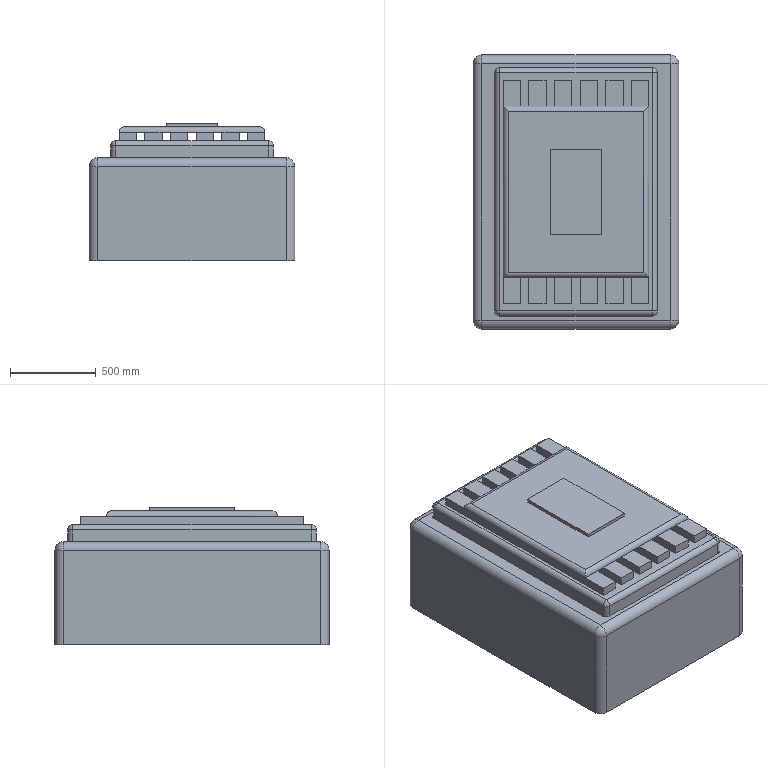Component | NX | 8_WORKBENCH | 10 solids | 84 faces | volume 1351351138 mm3 | plane 56 | cylinder 20 | sphere 8 | commonest cylinder face diameters 60 x12 100 x8